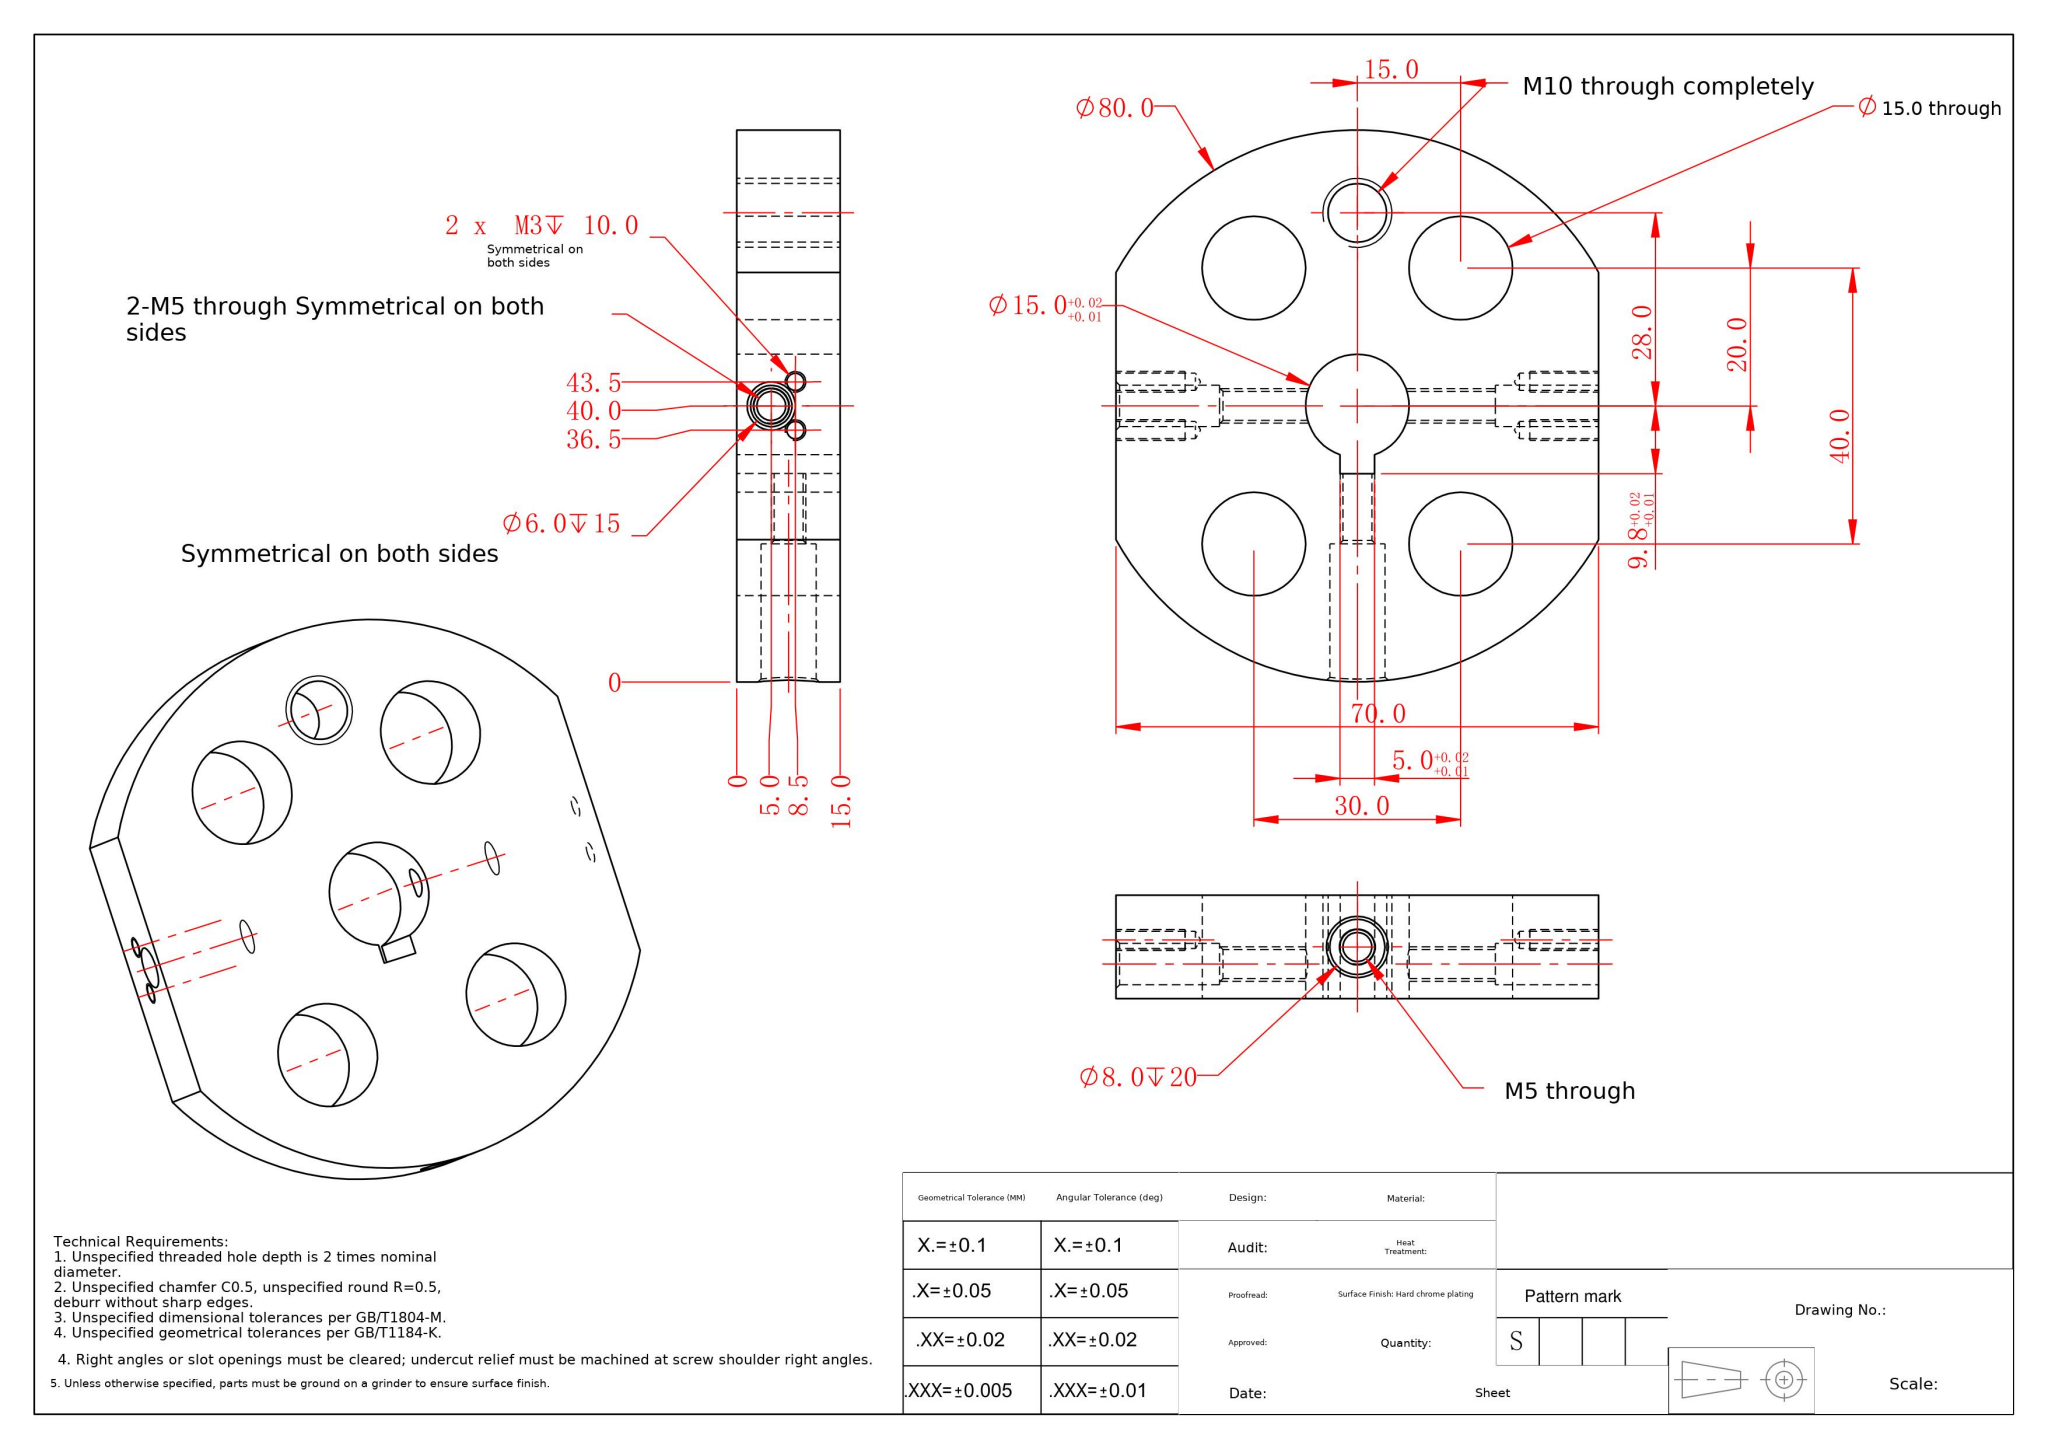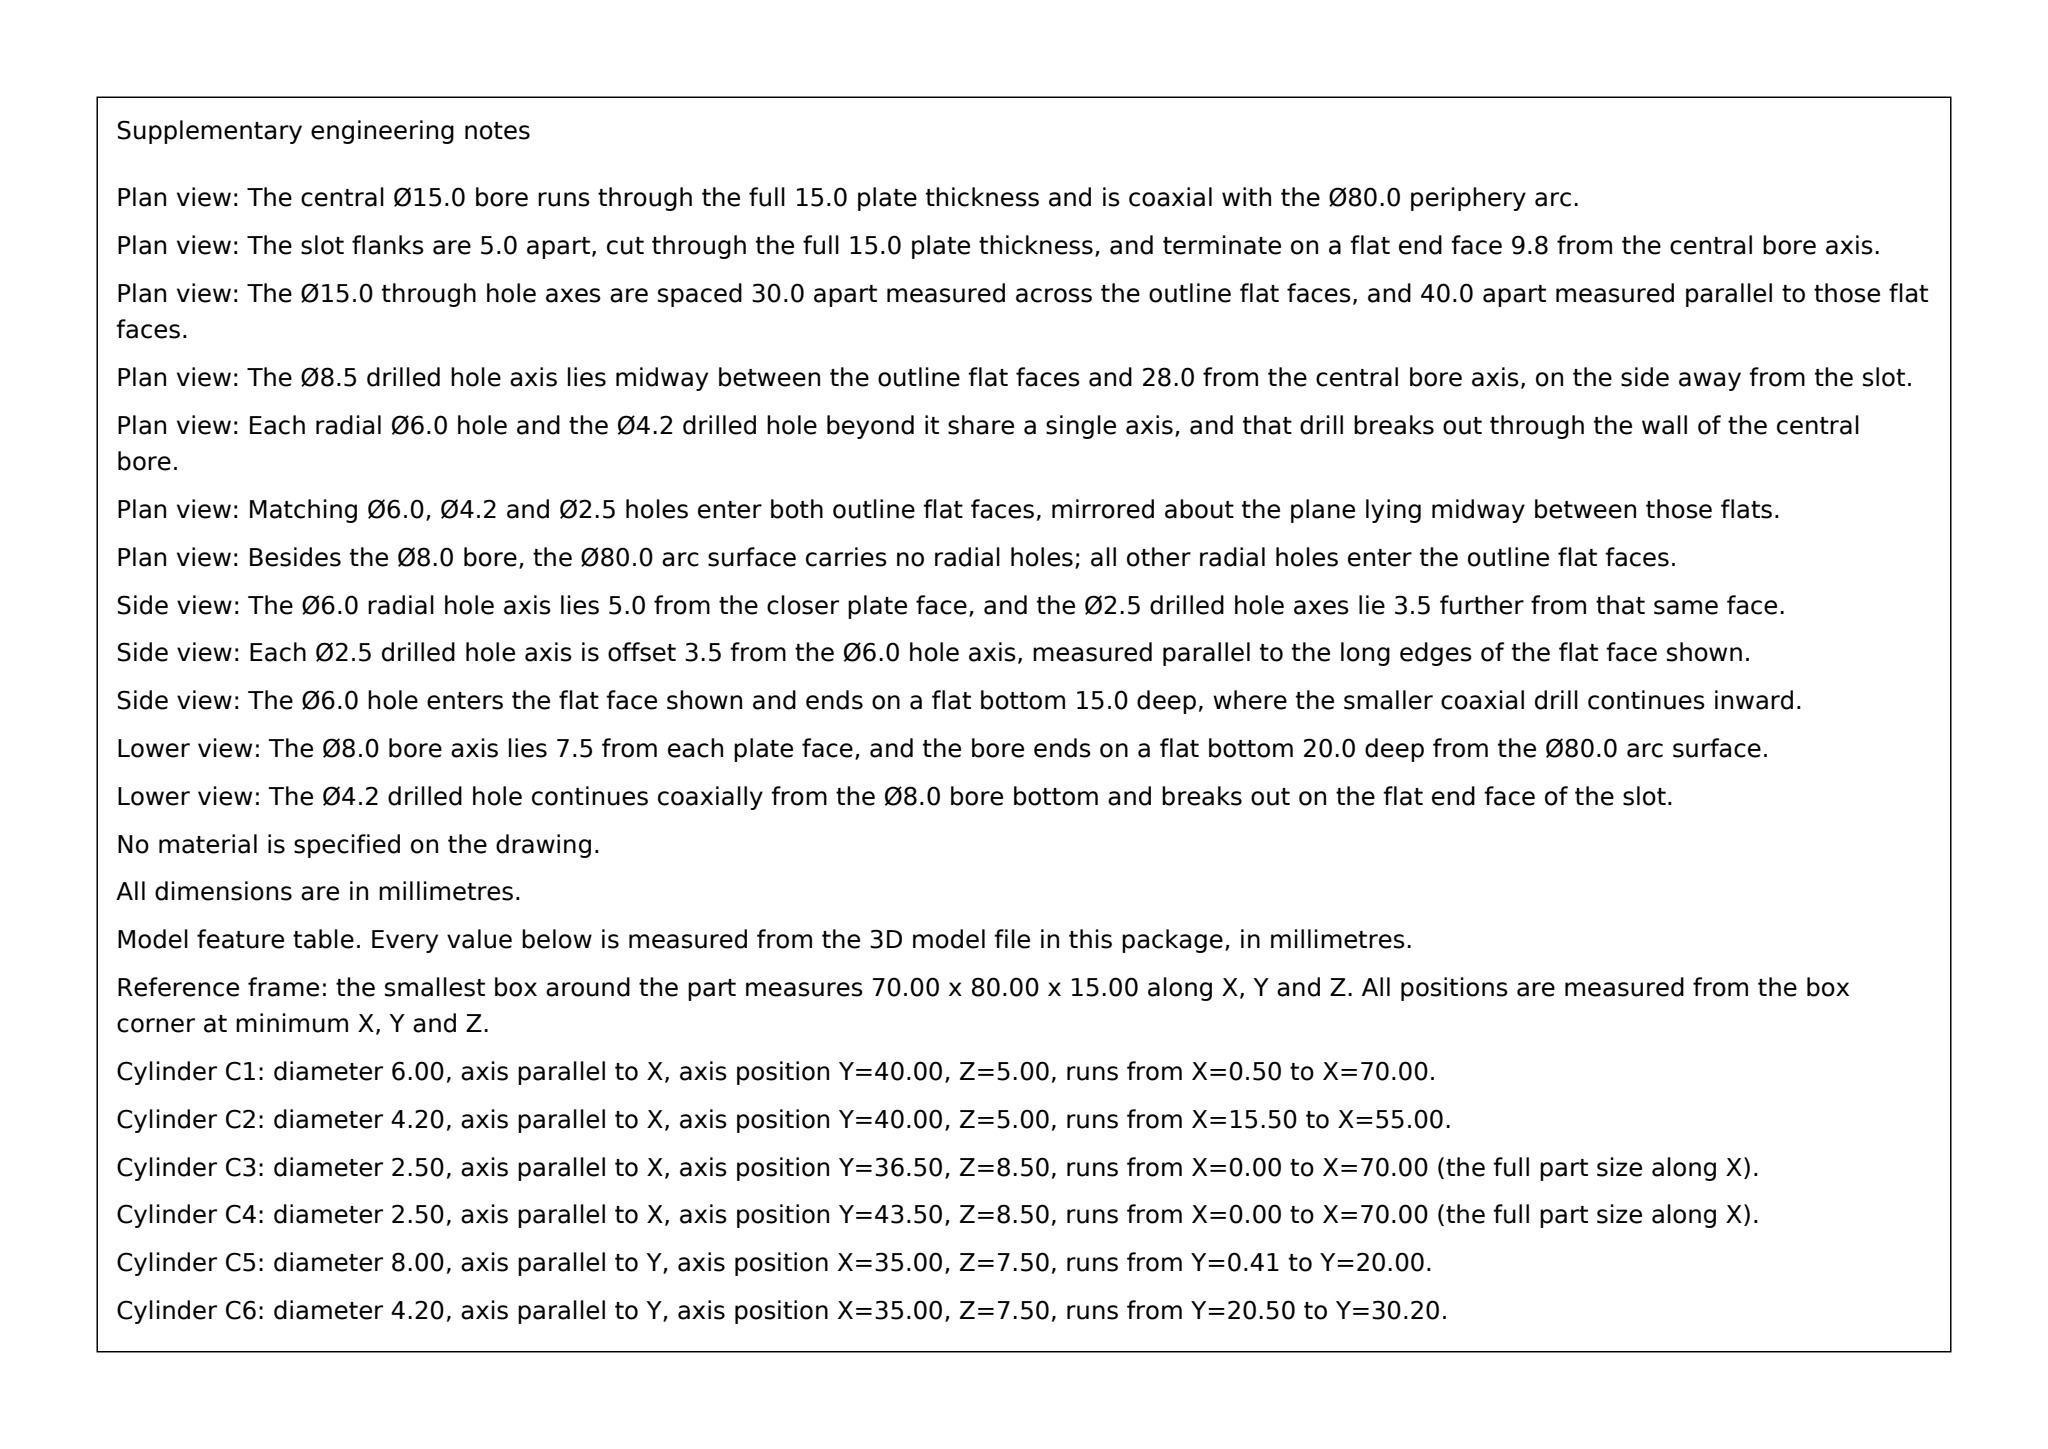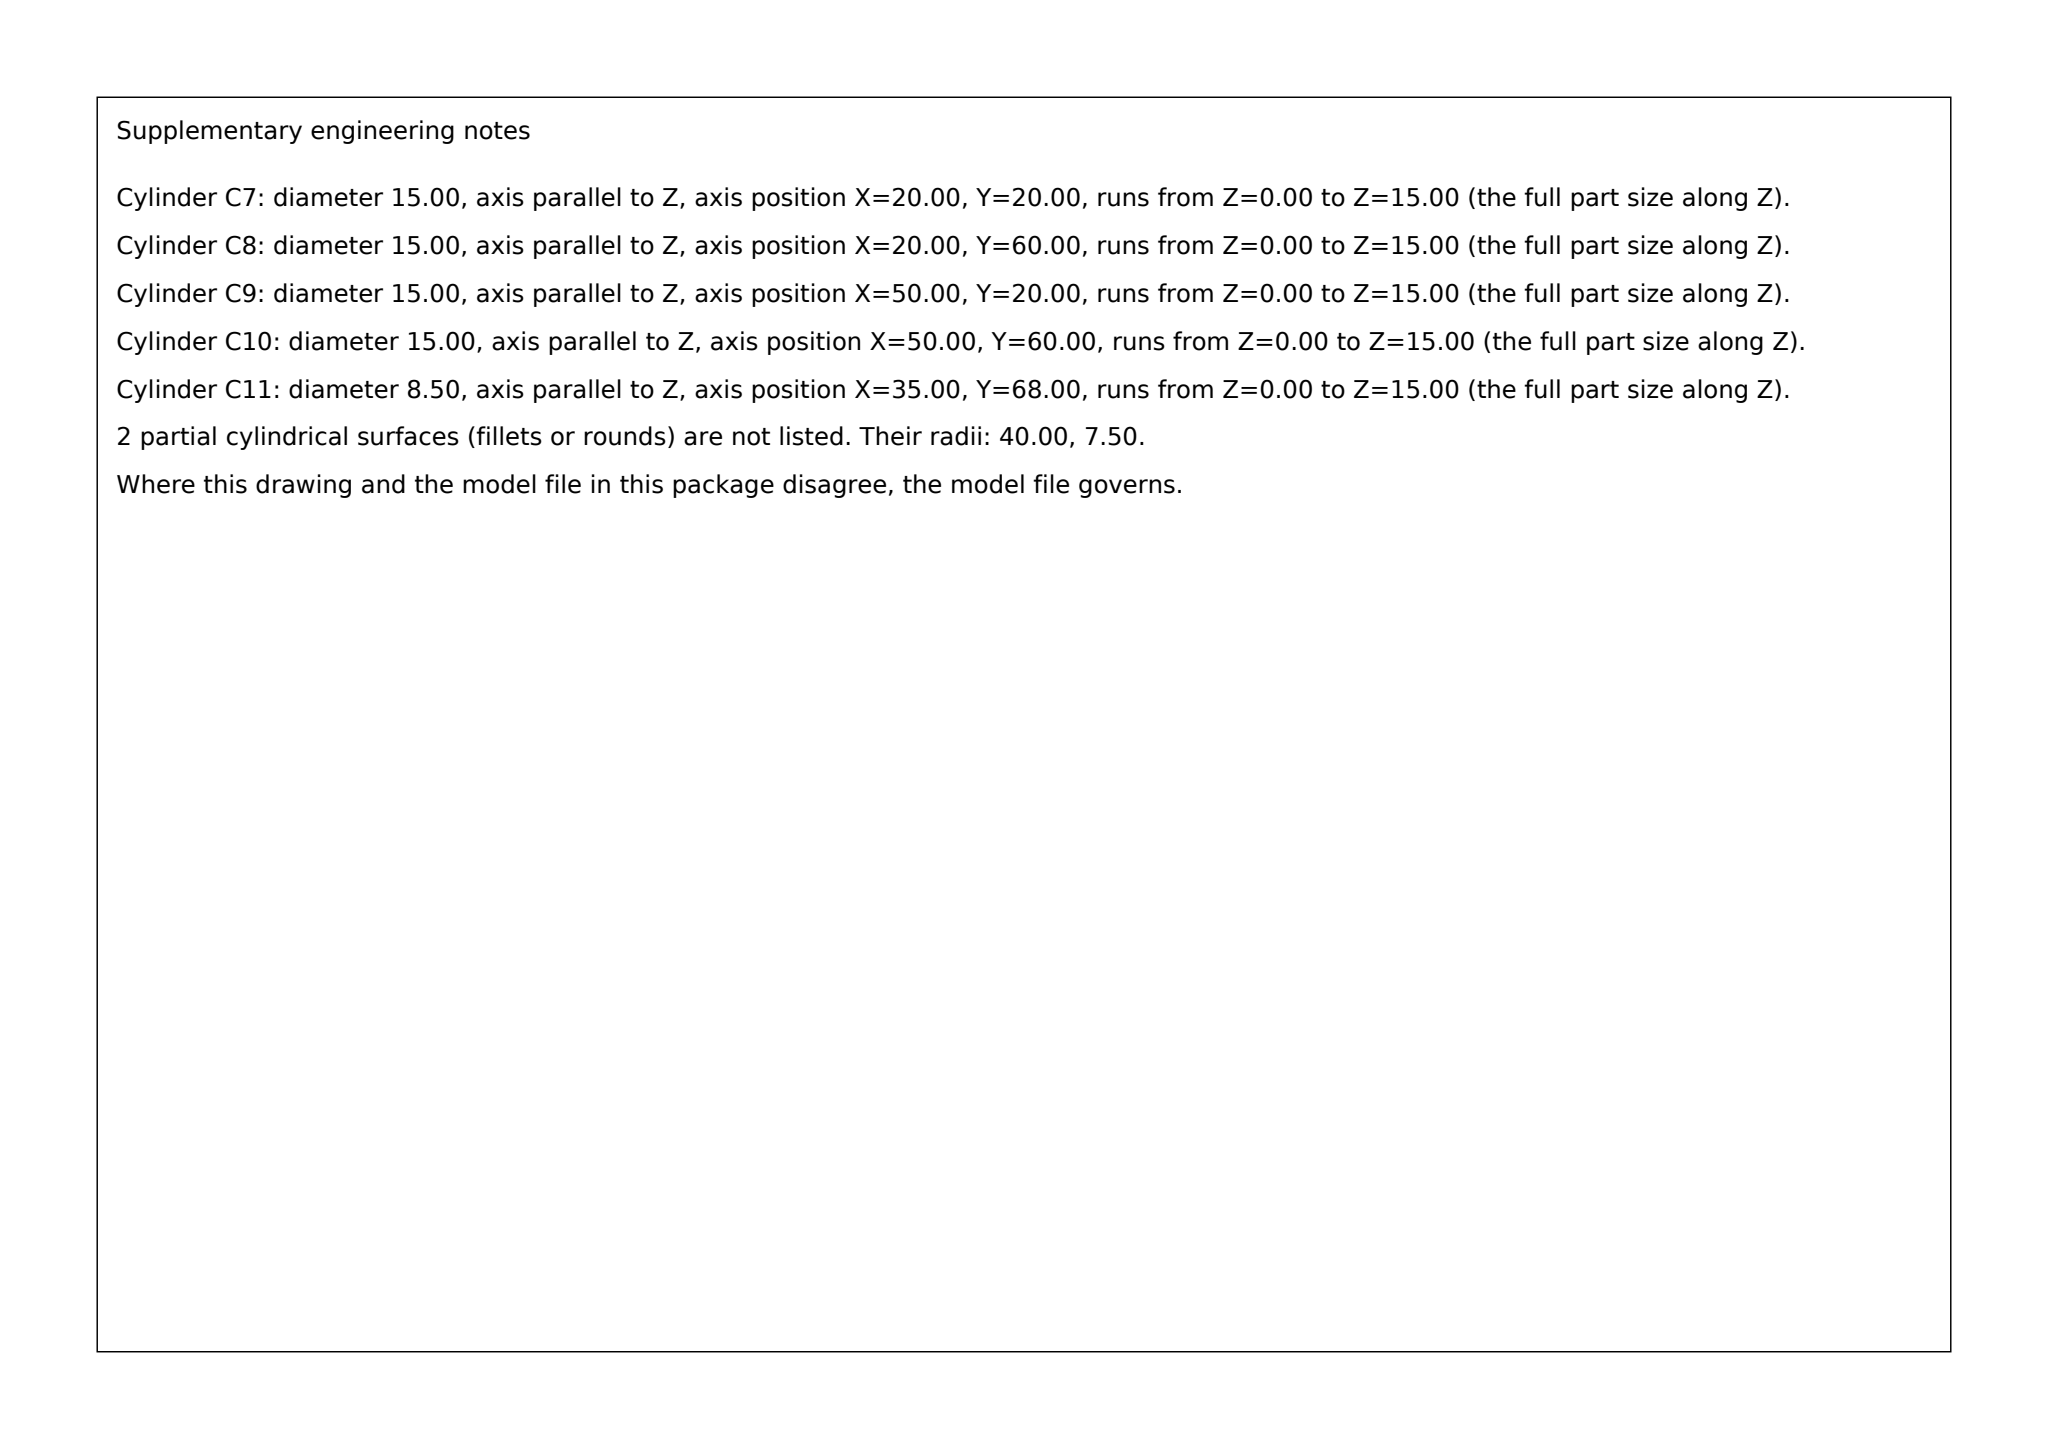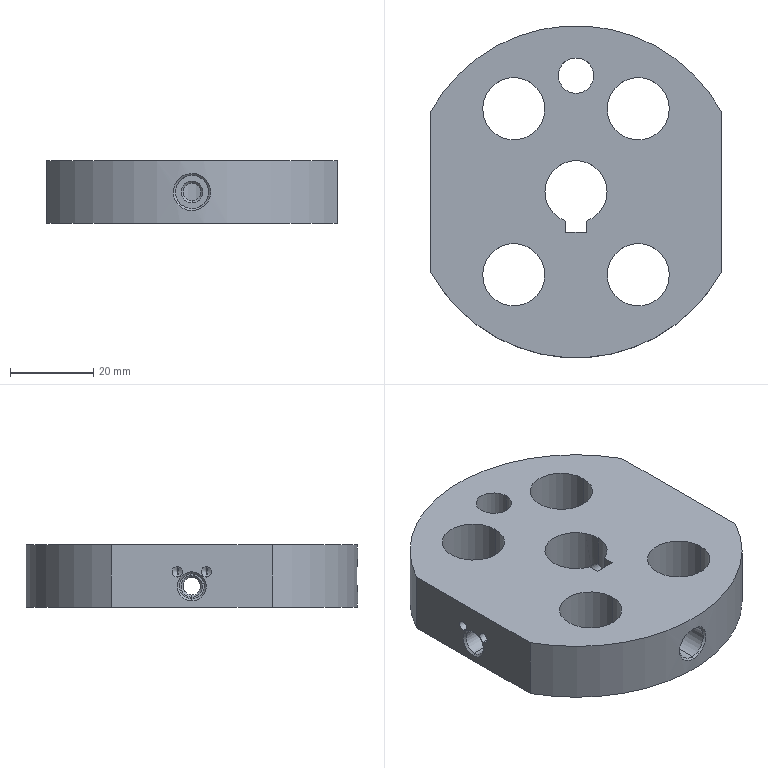Part | SolidWorks | mm | 1 solid | 61 faces | box 70 x 80 x 15 mm | volume 54606 mm3 | cylinder 35 | cone 14 | plane 10 | spline 2 | commonest cylinder face diameters 15 x11 2.5 x8 4.2 x6 6 x4 8 x2 8.5 x2 80 x2
Drawing notes:
STOCK: Ø80 DISC X 15 THK; 2X FLATS PARALLEL TO VERT CL, 35.0 EA SIDE, 70.0 ACROSS | from the solid: bbox 70.0(X) x 80.0(Y) x 15.0(Z); planes normal X at 0.0 & 70.0; Ø80 z-cyl CL x=35, L=15
Ø15 BORE CL AT X35.0 Y40.0, THRU 15 THK | from the solid: Ø15.0 z-axis cyl at (35,40), length 15.0
M10 THRU ON VERT CL, 28.0 ABOVE Ø15 BORE CL | from the solid: Ø8.5 z-axis thru hole at (35,68); Ø15 bore CL at (35,40) -> 28.0 in Y
SLOT BELOW Ø15 BORE: 5.0 WIDE, THRU 15 THK, END 9.8 BELOW BORE CL | from the solid: planes x=32.5 & x=37.5 (5.0 wide), y=30.2 end (40.0-30.2=9.8), thru z=0-15
2X SIDE HOLES ON HORIZ CL: Ø6.0 DP 15 + M5 THRU, 5.0 UP FROM BOT FACE | from the solid: Ø6.0 x-axis at y=40,z=5.0 to planes x=15.0/x=55.0; Ø4.2 x-axis thru on same axis
2X Ø8.0 DP 20 + M5 THRU ON VERT CL, 7.5 UP FROM BOT FACE | from the solid: Ø8.0 y-axis holes at (x=35,z=7.5) L=19.59, 2 off; Ø4.2 y-axis on same axis
4X M3 DP 10, 2X EA SIDE, AT Y36.5 & Y43.5, 8.5 UP FROM BOT FACE | from the solid: Ø2.5 x-axis holes at (y=36.5,z=8.5) and (y=43.5,z=8.5), 11.5 deep, 4 total